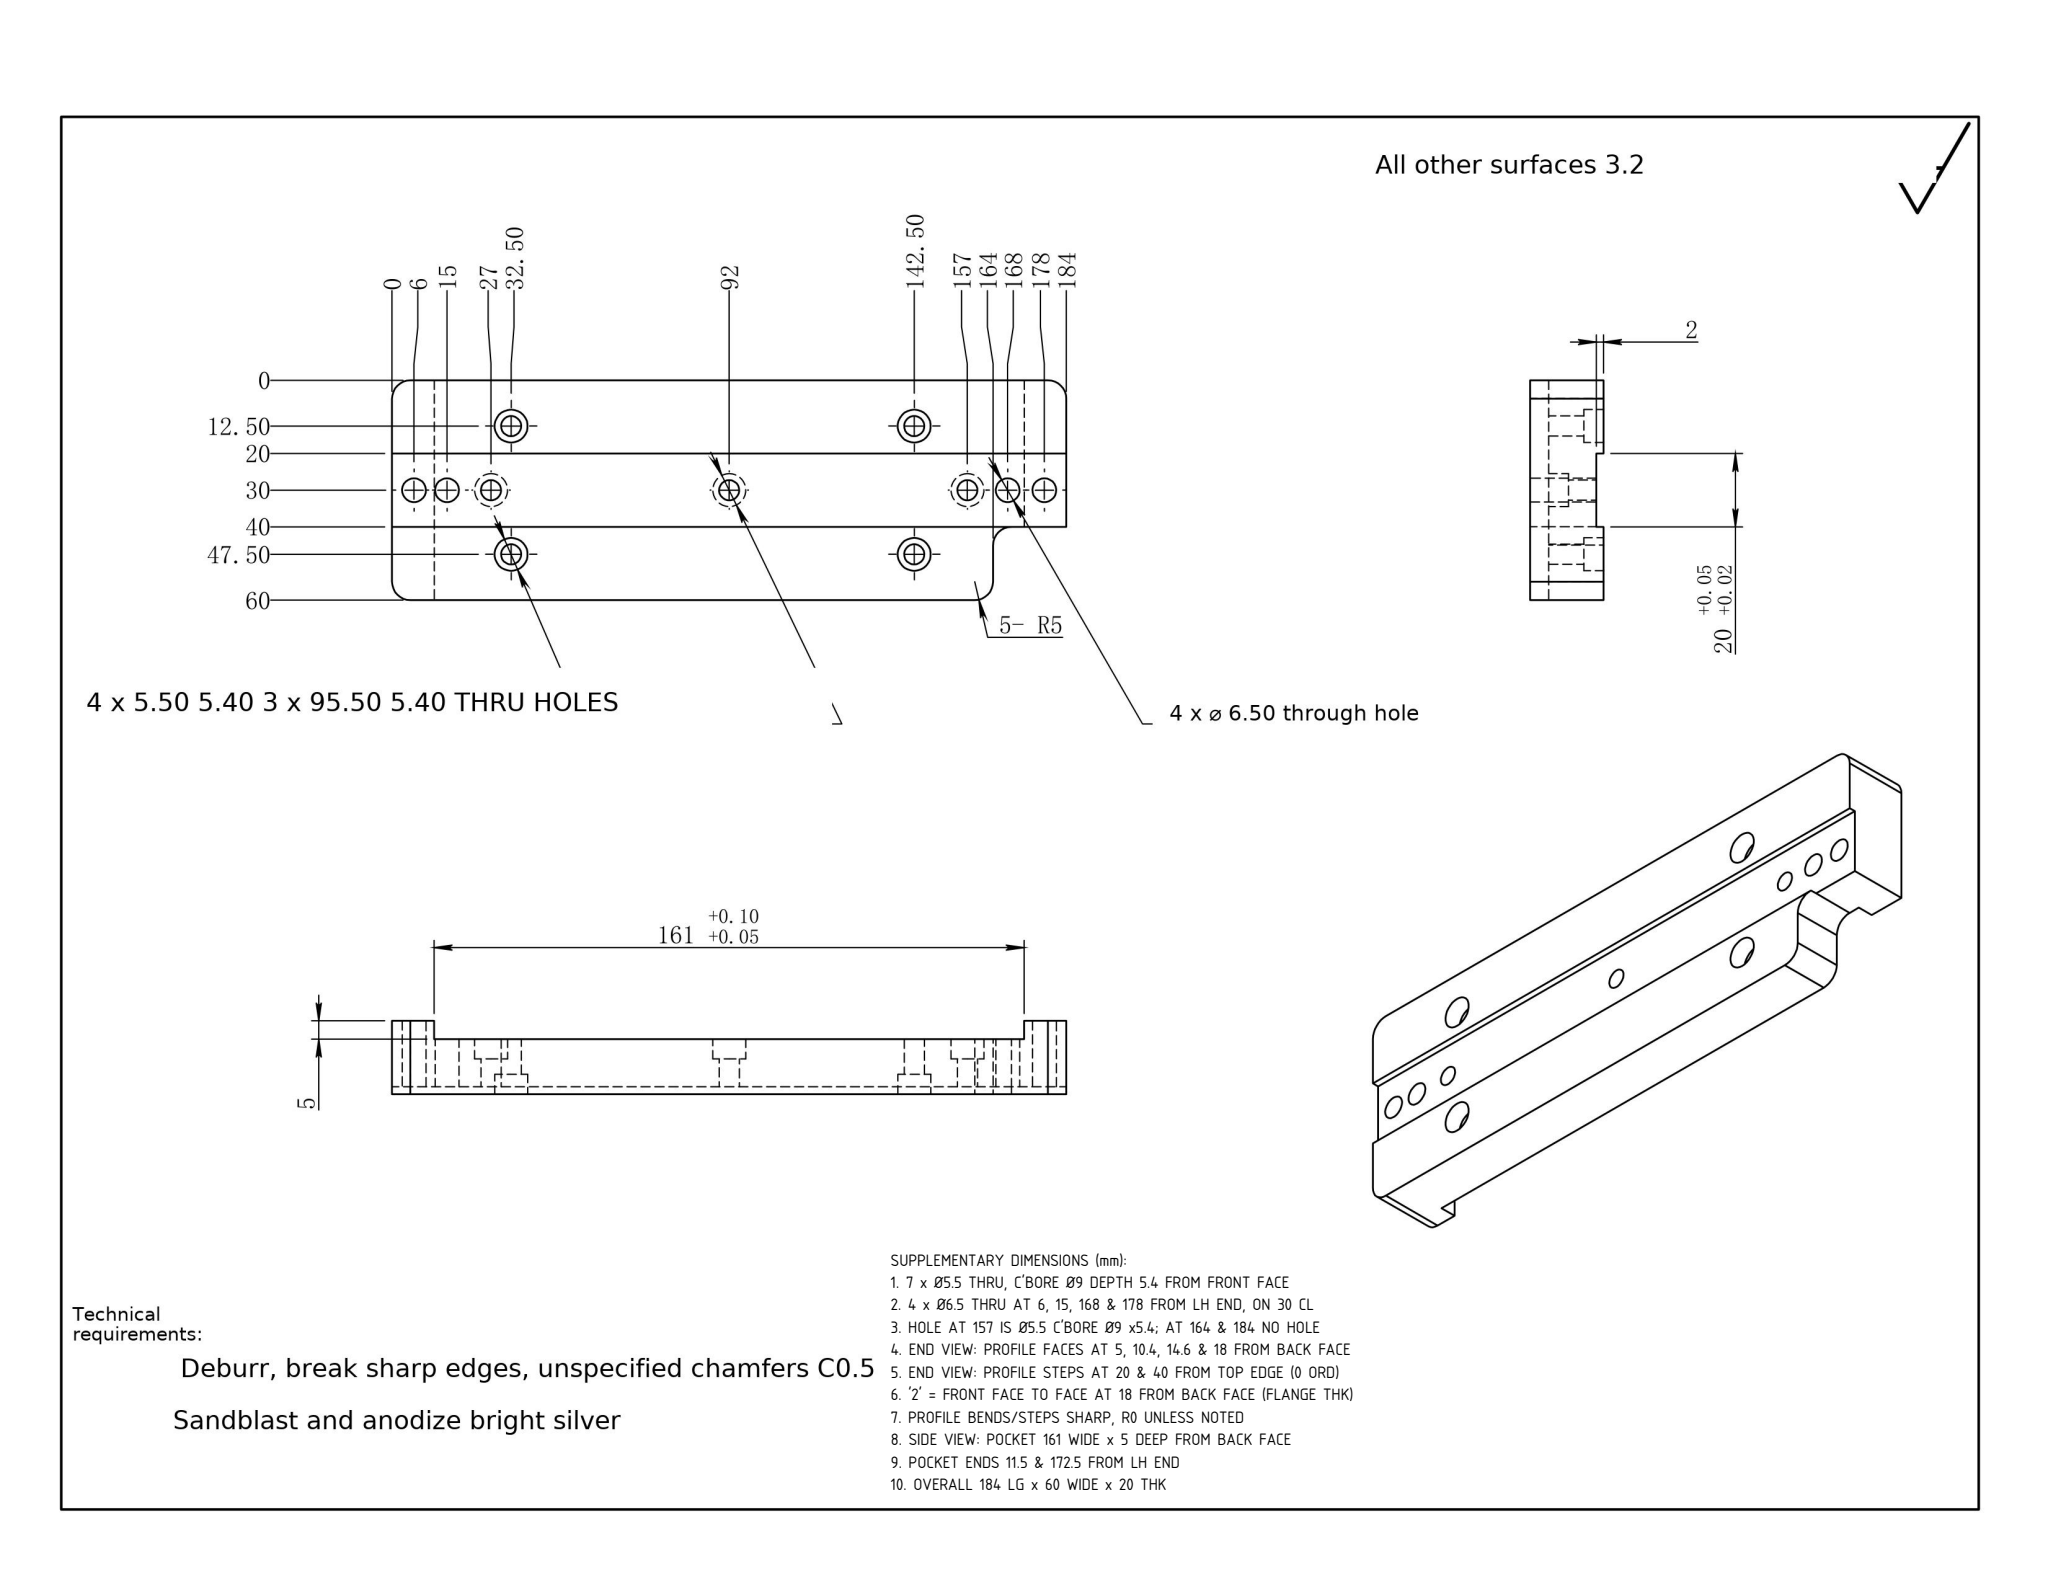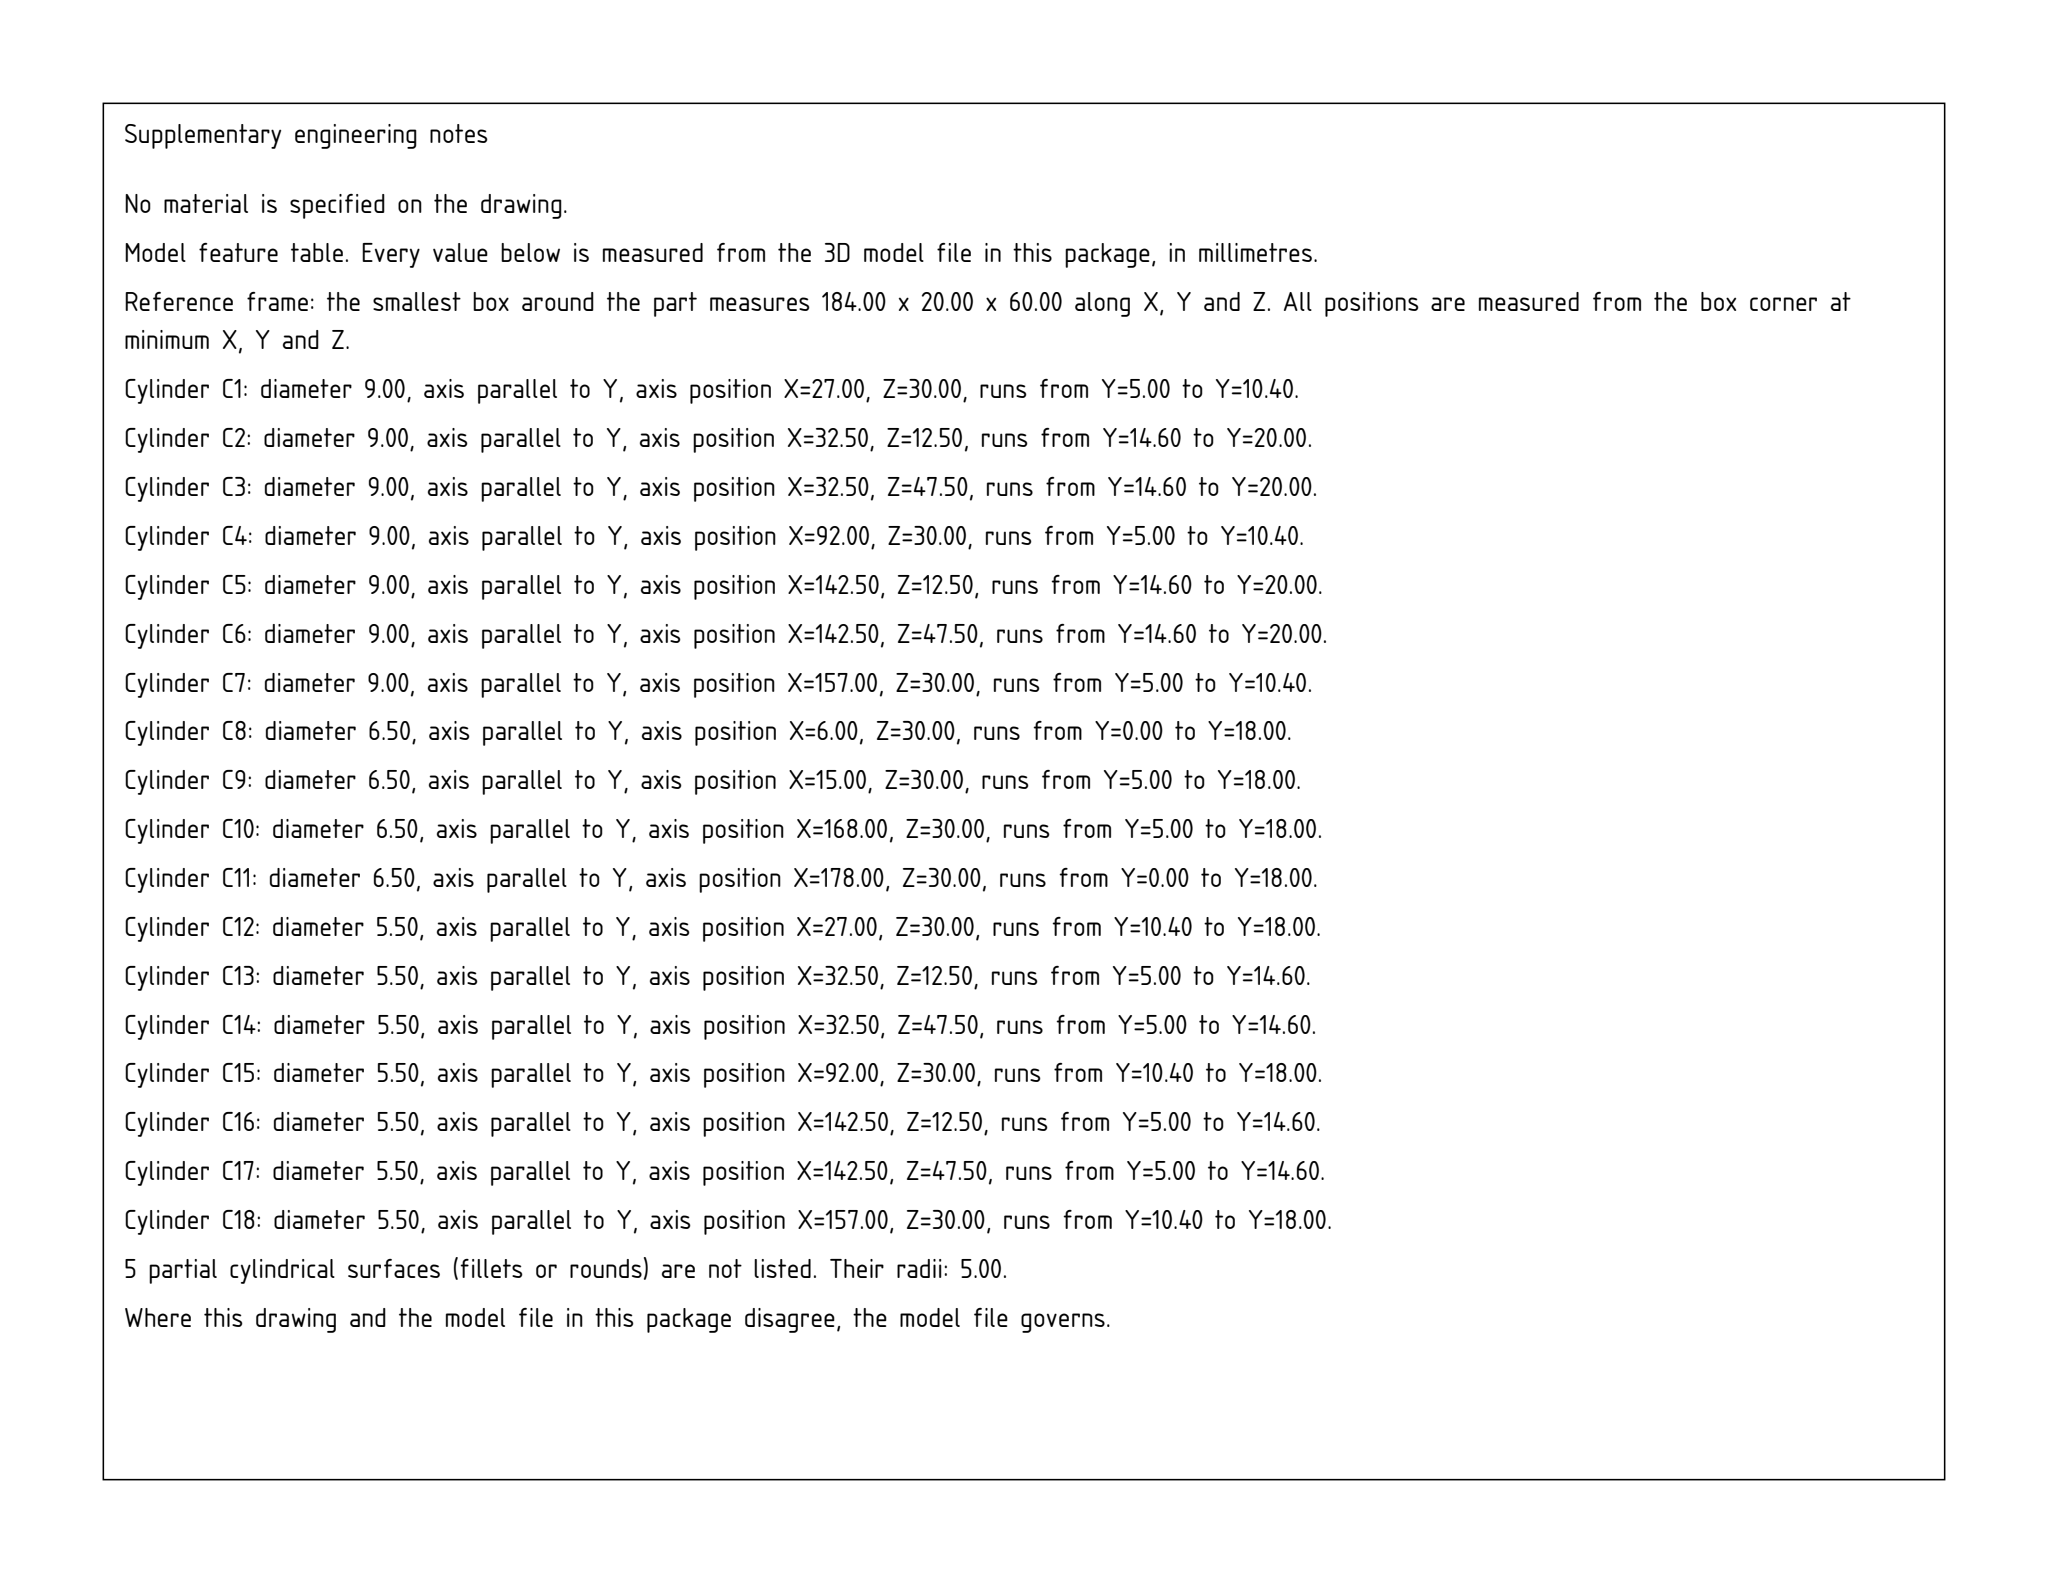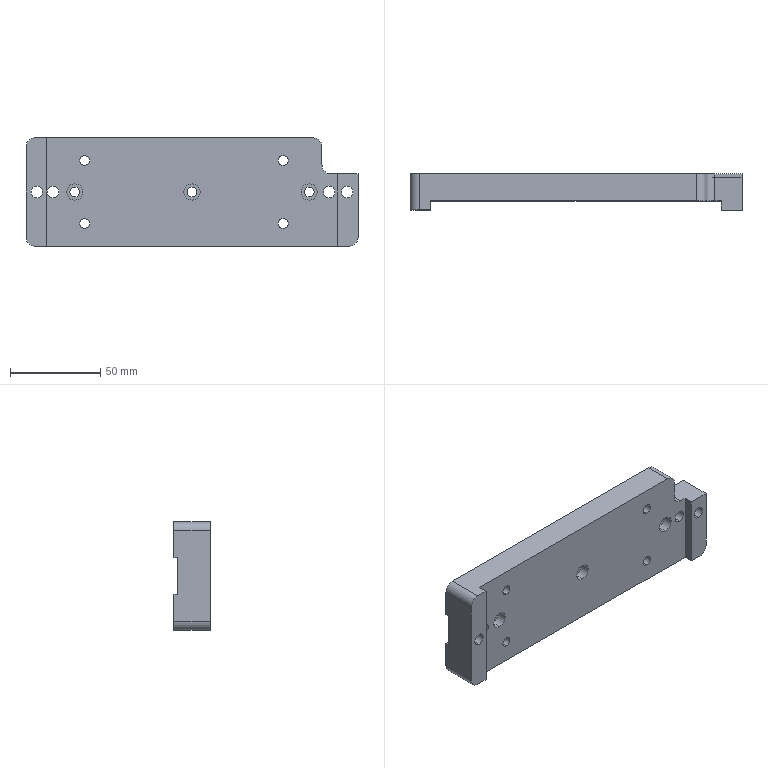Part | SolidWorks | mm | 1 solid | 64 faces | box 184 x 20 x 60 mm | volume 151752 mm3 | cylinder 41 | plane 23 | commonest cylinder face diameters 9 x14 5.5 x14 6.5 x8 10 x5
build123d program:
from build123d import *

# Parameters (mm, degrees)
SKETCH1_W                                       = 184
SKETCH1_H                                       = 60
BOSS_EXTRUDE1_DEPTH                             = 20
SKETCH2_W                                       = 161
SKETCH2_H                                       = 10
CUT_EXTRUDE1_DEPTH                              = 112.642
M5_HEX_SOCKET_HEAD_CAP_SCREW_CBORE1_D           = 5.5
M5_HEX_SOCKET_HEAD_CAP_SCREW_CBORE1_CBORE_D     = 9
M5_HEX_SOCKET_HEAD_CAP_SCREW_CBORE1_CBORE_DEPTH = 5.4
M5_HEX_SOCKET_HEAD_CAP_SCREW_CBORE3_D           = 5.5
M5_HEX_SOCKET_HEAD_CAP_SCREW_CBORE3_CBORE_D     = 9
M5_HEX_SOCKET_HEAD_CAP_SCREW_CBORE3_CBORE_DEPTH = 5.4
FILLET1_R                                       = 5
CUT_EXTRUDE2_DEPTH                              = 99.813
FILLET2_R                                       = 5
SKETCH12_W                                      = 20
SKETCH12_H                                      = 21.34
CUT_EXTRUDE3_DEPTH                              = 188.499
F_6_5_6_5_DIAMETER_HOLE1_D                      = 6.5


with BuildPart() as part:
    # Sketch1 → Boss-Extrude1 (new body)
    with BuildSketch(Plane(origin=(0, 0, 0), x_dir=(1, 0, 0), z_dir=(0, 1, 0))):
        Rectangle(SKETCH1_W, SKETCH1_H)
    extrude(amount=BOSS_EXTRUDE1_DEPTH)

    # Sketch2 → Cut-Extrude1 (cut, through all)
    with BuildSketch(Plane.XY.offset(30)):
        Rectangle(SKETCH2_W, SKETCH2_H)
    extrude(amount=-CUT_EXTRUDE1_DEPTH, mode=Mode.SUBTRACT)

    # M5 Hex Socket Head Cap Screw CBORE1 (through all)
    with Locations(Plane(origin=(0, 20, 0), x_dir=(1, 0, 0), z_dir=(0, 1, 0))):
        with Locations((-59.5, 17.5), (-59.5, -17.5), (50.5, -17.5), (50.5, 17.5)):
            CounterBoreHole(M5_HEX_SOCKET_HEAD_CAP_SCREW_CBORE1_D / 2, M5_HEX_SOCKET_HEAD_CAP_SCREW_CBORE1_CBORE_D / 2, M5_HEX_SOCKET_HEAD_CAP_SCREW_CBORE1_CBORE_DEPTH)

    # M5 Hex Socket Head Cap Screw CBORE3 (through all)
    with Locations(Plane(origin=(0, 5, 0), x_dir=(-1, 0, 0), z_dir=(0, -1, 0))):
        with Locations((65, 0), (-65, 0), (0, 0)):
            CounterBoreHole(M5_HEX_SOCKET_HEAD_CAP_SCREW_CBORE3_D / 2, M5_HEX_SOCKET_HEAD_CAP_SCREW_CBORE3_CBORE_D / 2, M5_HEX_SOCKET_HEAD_CAP_SCREW_CBORE3_CBORE_DEPTH)

    # Fillet1
    fillet1_edges = [part.edges().sort_by_distance(p)[0] for p in [
        (92, 10, 30),
        (-92, 10, 30),
        (-92, 10, -30),
        (92, 10, -30),
    ]]
    fillet(fillet1_edges, radius=FILLET1_R)

    # Sketch11 → Cut-Extrude2 (cut, through all)
    with BuildSketch(Plane(origin=(0, 20, 0), x_dir=(1, 0, 0), z_dir=(0, 1, 0))):
        with BuildLine():
            Line((92, -10), (77, -10))
            ThreePointArc((77, -10), (73.464, -11.464), (72, -15))
            Line((72, -15), (72, -30))
            Line((72, -30), (92, -30))
            Line((92, -30), (92, -10))
        make_face()
    extrude(amount=-CUT_EXTRUDE2_DEPTH, mode=Mode.SUBTRACT)

    # Fillet2
    fillet2_edges = [part.edges().sort_by_distance(p)[0] for p in [
        (72, 12.5, 30),
    ]]
    fillet(fillet2_edges, radius=FILLET2_R)

    # Sketch12 → Cut-Extrude3 (cut, through all)
    with BuildSketch(Plane(origin=(92, 0, 0), x_dir=(0, 0, -1), z_dir=(1, 0, 0))):
        with Locations((0, 28.67)):
            Rectangle(SKETCH12_W, SKETCH12_H)
    extrude(amount=-CUT_EXTRUDE3_DEPTH, mode=Mode.SUBTRACT)

    # 6.5 _6.5_ Diameter Hole1 (through all)
    with Locations(Plane(origin=(0, 20, 0), x_dir=(1, 0, 0), z_dir=(0, 1, 0))):
        with Locations((-77, 0), (-86, 0), (76, 0), (86, 0)):
            Hole(F_6_5_6_5_DIAMETER_HOLE1_D / 2)


solid = part.part